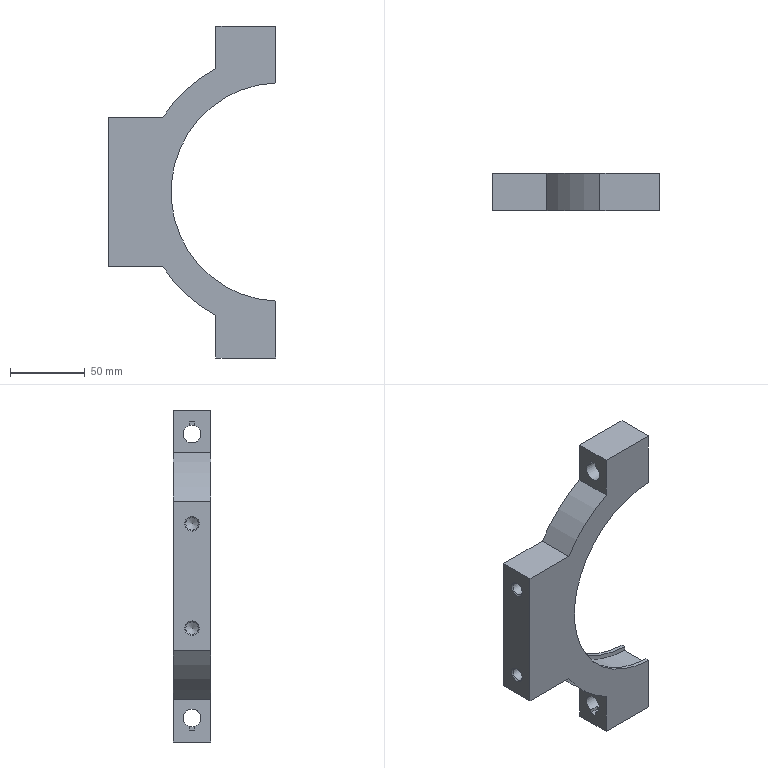Component | NX | STRAP_2 | 1 solid | 34 faces | volume 211145 mm3 | plane 21 | cylinder 9 | cone 4 | commonest cylinder face diameters 146 x2 186 x2 12 x2 8.5 x2 152 x1